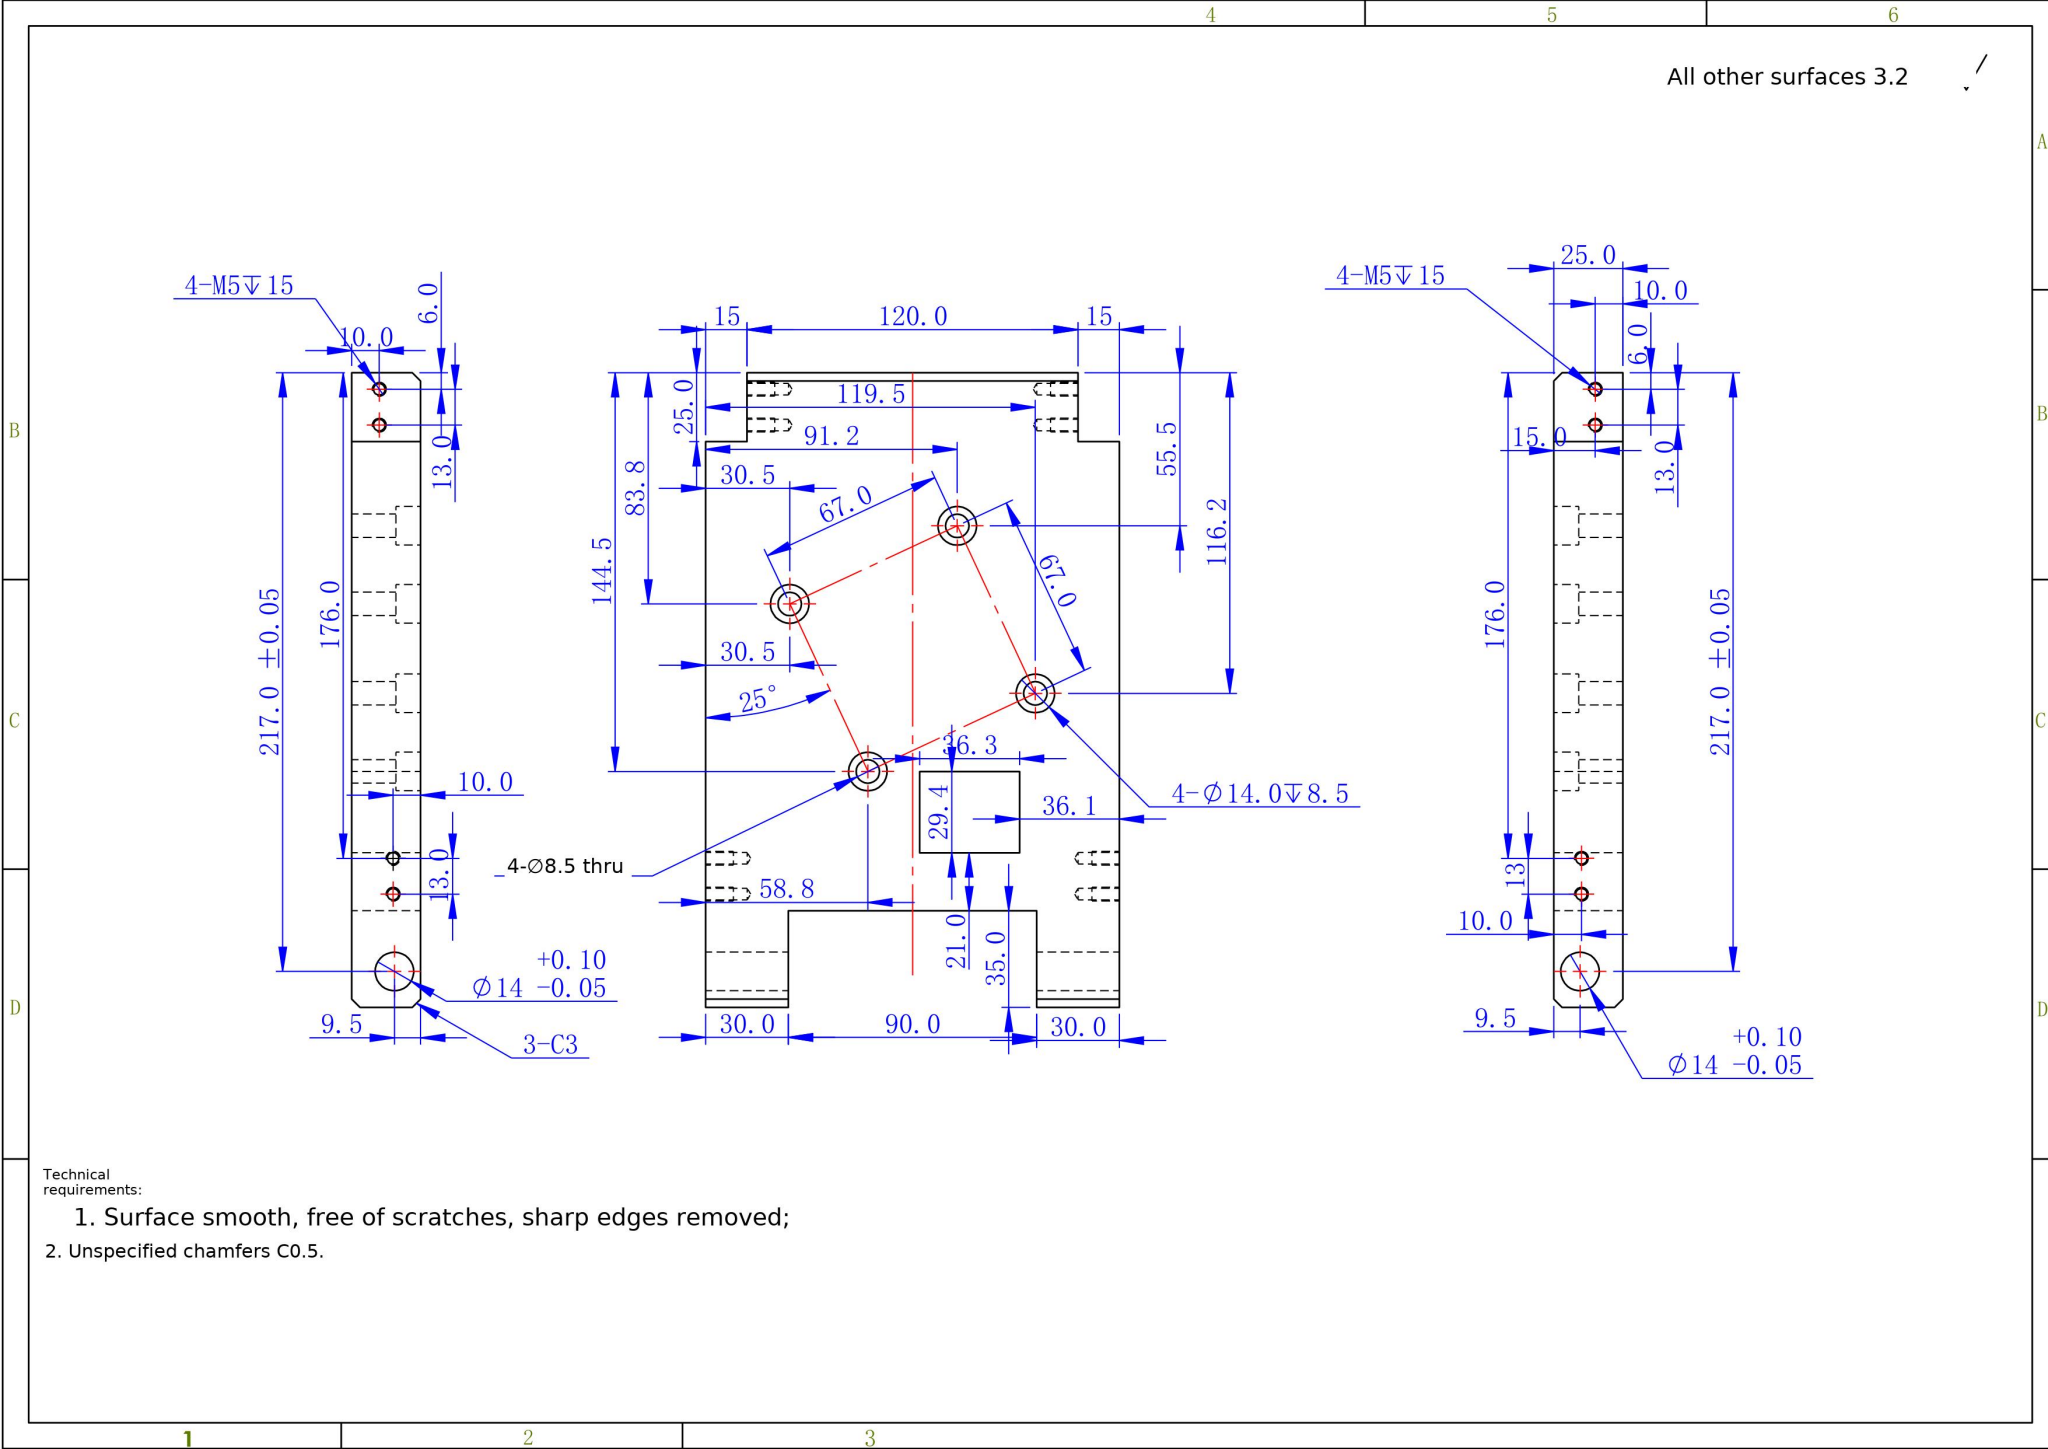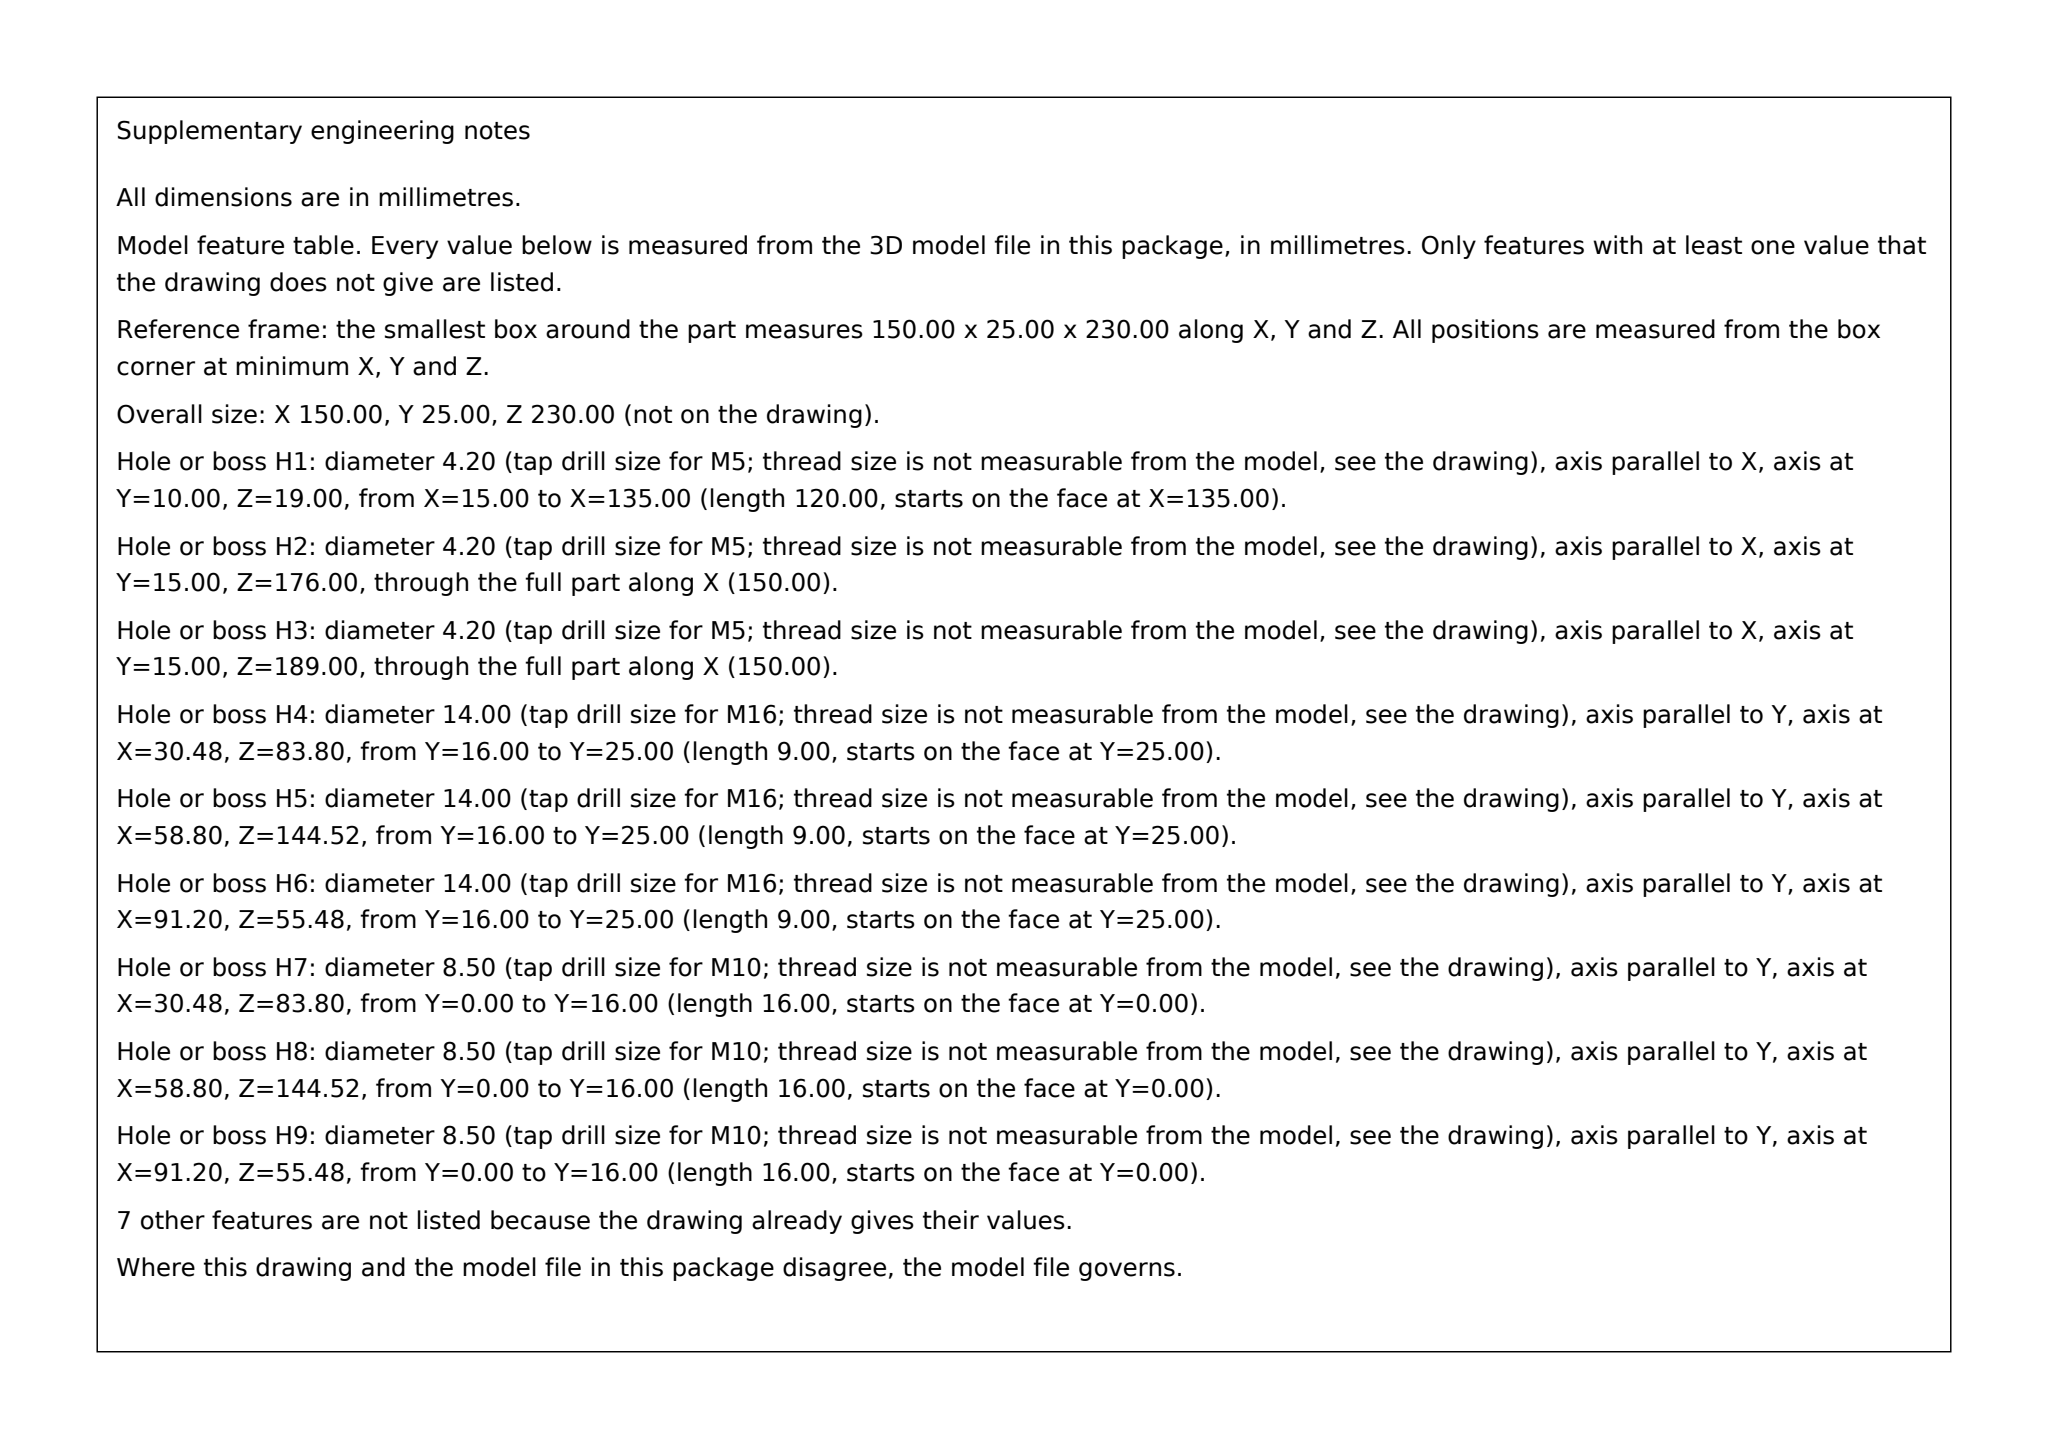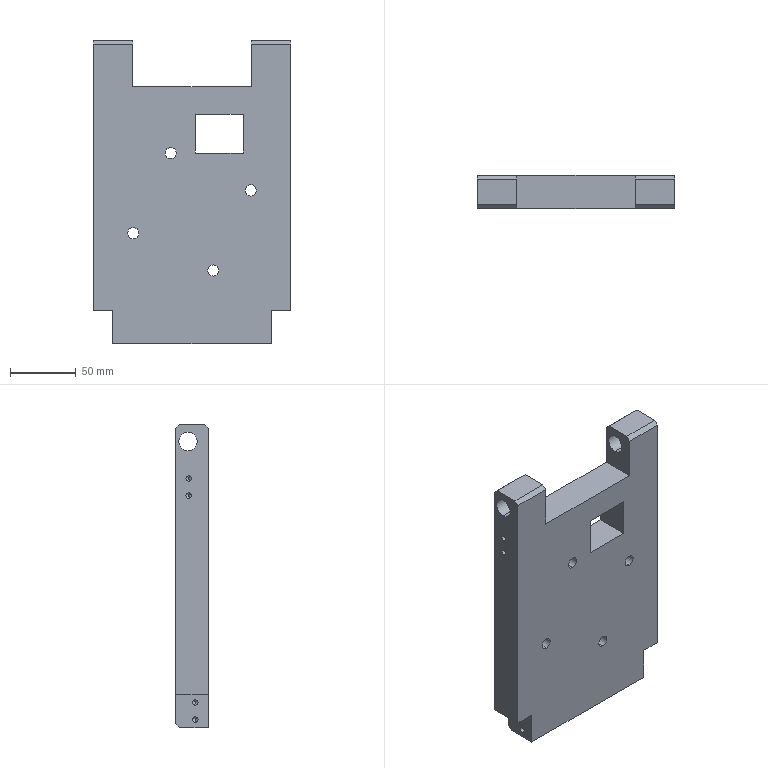Part | SolidWorks | mm | 1 solid | 79 faces | box 150 x 25 x 230 mm | volume 717106 mm3 | cylinder 36 | plane 27 | cone 16 | commonest cylinder face diameters 4.2 x16 14 x12 8.5 x8